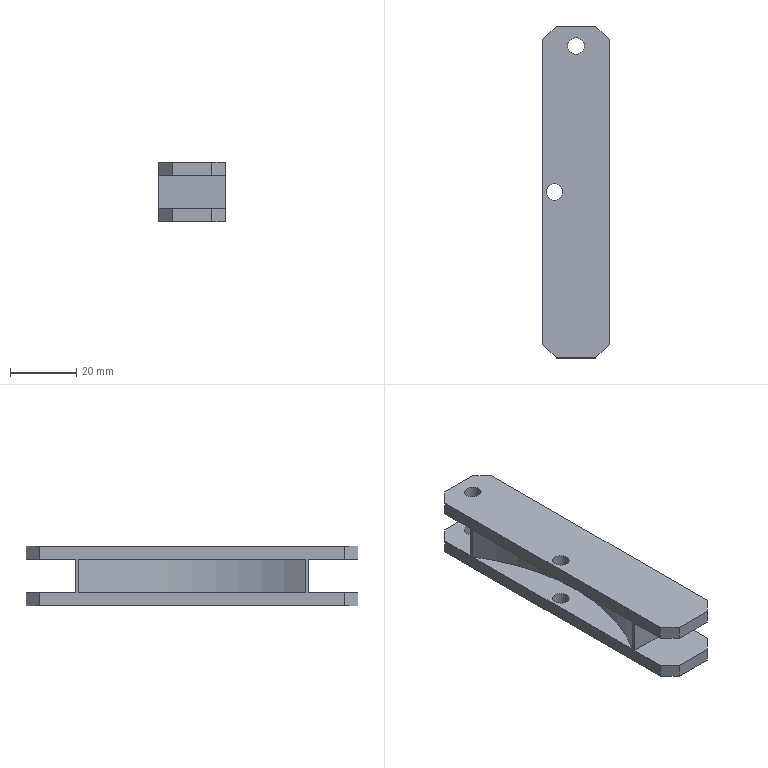Component | NX | HINGE_CLAMP_PLATE | 1 solid | 29 faces | volume 24811 mm3 | plane 24 | cylinder 5 | commonest cylinder face diameters 5 x4 126 x1